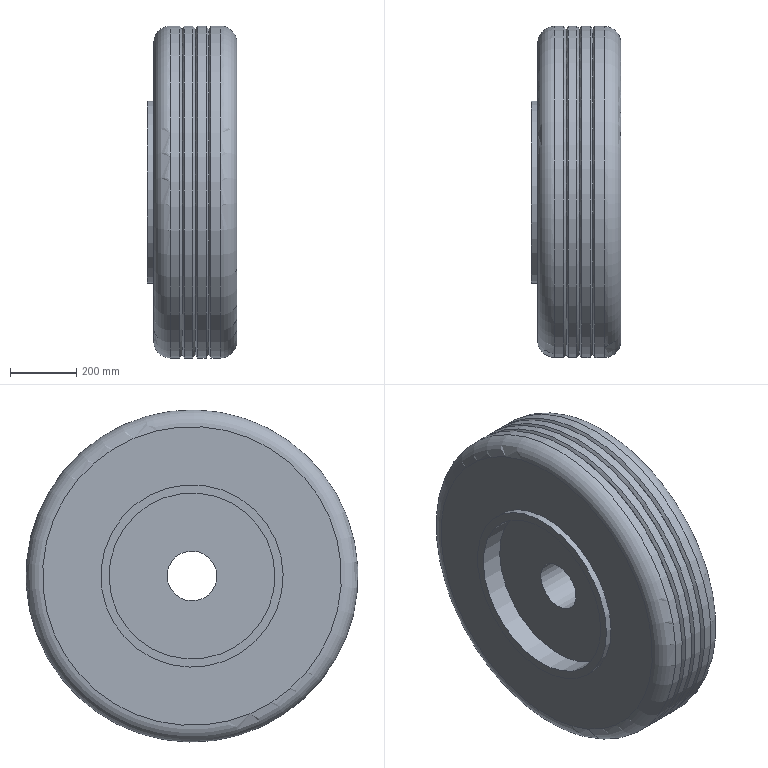Component | NX | WHEEL | 1 solid | 19 faces | box 270 x 1000 x 1000 mm | volume 179843524 mm3 | cylinder 7 | cone 6 | plane 4 | torus 2 | commonest cylinder face diameters 1000 x4 150 x1 500 x1 549 x1
STEP:
#1=CARTESIAN_POINT('',(0.,0.,0.));
#2=DIRECTION('',(0.,0.,1.));
#3=DIRECTION('',(1.,0.,0.));
#4=AXIS2_PLACEMENT_3D('',#1,#2,#3);
#5=CARTESIAN_POINT('',(283.134,-1440.025,-27.809));
#6=VERTEX_POINT('',#5);
#7=CARTESIAN_POINT('',(283.134,-1370.568,0.4891));
#8=DIRECTION('',(1.,0.,0.));
#9=DIRECTION('',(0.,-0.9261,-0.3773));
#10=AXIS2_PLACEMENT_3D('',#7,#8,#9);
#11=CIRCLE('',#10,75.);
#12=CARTESIAN_POINT('',(283.134,-1200.783,-416.252));
#13=DIRECTION('',(-1.,0.,0.));
#14=DIRECTION('',(0.,0.9261,0.3773));
#15=AXIS2_PLACEMENT_3D('',#12,#13,#14);
#16=PLANE('',#15);
#17=CARTESIAN_POINT('',(-75.,-450.));
#18=CARTESIAN_POINT('',(-75.,-320.096));
#19=CARTESIAN_POINT('',(37.5,-385.048));
#20=CARTESIAN_POINT('',(150.,-450.));
#21=CARTESIAN_POINT('',(37.5,-514.952));
#22=CARTESIAN_POINT('',(-75.,-579.904));
#23=CARTESIAN_POINT('',(-75.,-450.));
#24=(BOUNDED_CURVE()B_SPLINE_CURVE(2,(#17,#18,#19,#20,#21,#22,#23),.UNSPECIFIED.,.T.,.F.)B_SPLINE_CURVE_WITH_KNOTS((1,2,2,2,2,1),(-2.094,0.,2.094,4.189,6.283,8.378),.UNSPECIFIED.)CURVE()GEOMETRIC_REPRESENTATION_ITEM()RATIONAL_B_SPLINE_CURVE((1.,0.5,1.,0.5,1.,0.5,1.))REPRESENTATION_ITEM(''));
#25=(GEOMETRIC_REPRESENTATION_CONTEXT(2)PARAMETRIC_REPRESENTATION_CONTEXT()REPRESENTATION_CONTEXT('',''));
#26=DEFINITIONAL_REPRESENTATION('',(#24),#25);
#27=PCURVE('',#16,#26);
#28=CARTESIAN_POINT('',(158.134,-1370.568,0.4891));
#29=DIRECTION('',(1.,0.,0.));
#30=DIRECTION('',(0.,-0.9261,-0.3773));
#31=AXIS2_PLACEMENT_3D('',#28,#29,#30);
#32=CYLINDRICAL_SURFACE('',#31,75.);
#33=CARTESIAN_POINT('',(0.,125.));
#34=DIRECTION('',(1.,0.));
#35=VECTOR('',#34,1.);
#36=LINE('',#33,#35);
#37=(GEOMETRIC_REPRESENTATION_CONTEXT(2)PARAMETRIC_REPRESENTATION_CONTEXT()REPRESENTATION_CONTEXT('',''));
#38=DEFINITIONAL_REPRESENTATION('',(#36),#37);
#39=PCURVE('',#32,#38);
#40=SURFACE_CURVE('',#11,(#27,#39),.PCURVE_S1.);
#41=EDGE_CURVE('',#6,#6,#40,.T.);
#42=ORIENTED_EDGE('',*,*,#41,.F.);
#43=EDGE_LOOP('',(#42));
#44=FACE_BOUND('',#43,.T.);
#45=CARTESIAN_POINT('',(283.134,-1787.309,-169.297));
#46=VERTEX_POINT('',#45);
#47=CARTESIAN_POINT('',(283.134,-1370.568,0.4891));
#48=DIRECTION('',(1.,0.,0.));
#49=DIRECTION('',(0.,-0.9261,-0.3773));
#50=AXIS2_PLACEMENT_3D('',#47,#48,#49);
#51=CIRCLE('',#50,450.);
#52=CARTESIAN_POINT('',(-450.,-450.));
#53=CARTESIAN_POINT('',(-450.,329.423));
#54=CARTESIAN_POINT('',(225.,-60.289));
#55=CARTESIAN_POINT('',(900.,-450.));
#56=CARTESIAN_POINT('',(225.,-839.711));
#57=CARTESIAN_POINT('',(-450.,-1229.423));
#58=CARTESIAN_POINT('',(-450.,-450.));
#59=(BOUNDED_CURVE()B_SPLINE_CURVE(2,(#52,#53,#54,#55,#56,#57,#58),.UNSPECIFIED.,.T.,.F.)B_SPLINE_CURVE_WITH_KNOTS((1,2,2,2,2,1),(-2.094,0.,2.094,4.189,6.283,8.378),.UNSPECIFIED.)CURVE()GEOMETRIC_REPRESENTATION_ITEM()RATIONAL_B_SPLINE_CURVE((1.,0.5,1.,0.5,1.,0.5,1.))REPRESENTATION_ITEM(''));
#60=(GEOMETRIC_REPRESENTATION_CONTEXT(2)PARAMETRIC_REPRESENTATION_CONTEXT()REPRESENTATION_CONTEXT('',''));
#61=DEFINITIONAL_REPRESENTATION('',(#59),#60);
#62=PCURVE('',#16,#61);
#63=CARTESIAN_POINT('',(233.134,-1370.568,0.4891));
#64=DIRECTION('',(1.,0.,0.));
#65=DIRECTION('',(0.,-0.9261,-0.3773));
#66=AXIS2_PLACEMENT_3D('',#63,#64,#65);
#67=TOROIDAL_SURFACE('',#66,450.,50.);
#68=CARTESIAN_POINT('',(0.,7.854));
#69=DIRECTION('',(1.,0.));
#70=VECTOR('',#69,1.);
#71=LINE('',#68,#70);
#72=(GEOMETRIC_REPRESENTATION_CONTEXT(2)PARAMETRIC_REPRESENTATION_CONTEXT()REPRESENTATION_CONTEXT('',''));
#73=DEFINITIONAL_REPRESENTATION('',(#71),#72);
#74=PCURVE('',#67,#73);
#75=SURFACE_CURVE('',#51,(#62,#74),.PCURVE_S1.);
#76=EDGE_CURVE('',#46,#46,#75,.T.);
#77=ORIENTED_EDGE('',*,*,#76,.T.);
#78=EDGE_LOOP('',(#77));
#79=FACE_BOUND('',#78,.T.);
#80=ADVANCED_FACE('',(#44,#79),#16,.F.);
#81=CARTESIAN_POINT('',(83.134,-1440.025,-27.809));
#82=VERTEX_POINT('',#81);
#83=CARTESIAN_POINT('',(83.134,-1370.568,0.4891));
#84=DIRECTION('',(1.,0.,0.));
#85=DIRECTION('',(0.,-0.9261,-0.3773));
#86=AXIS2_PLACEMENT_3D('',#83,#84,#85);
#87=CIRCLE('',#86,75.);
#88=CARTESIAN_POINT('',(0.,-75.));
#89=DIRECTION('',(1.,0.));
#90=VECTOR('',#89,1.);
#91=LINE('',#88,#90);
#92=(GEOMETRIC_REPRESENTATION_CONTEXT(2)PARAMETRIC_REPRESENTATION_CONTEXT()REPRESENTATION_CONTEXT('',''));
#93=DEFINITIONAL_REPRESENTATION('',(#91),#92);
#94=PCURVE('',#32,#93);
#95=CARTESIAN_POINT('',(83.134,-1342.271,-68.968));
#96=DIRECTION('',(1.,0.,0.));
#97=DIRECTION('',(0.,-0.9261,-0.3773));
#98=AXIS2_PLACEMENT_3D('',#95,#96,#97);
#99=PLANE('',#98);
#100=CARTESIAN_POINT('',(-0.,-75.));
#101=DIRECTION('',(1.,0.));
#102=AXIS2_PLACEMENT_2D('',#100,#101);
#103=CIRCLE('',#102,75.);
#104=(GEOMETRIC_REPRESENTATION_CONTEXT(2)PARAMETRIC_REPRESENTATION_CONTEXT()REPRESENTATION_CONTEXT('',''));
#105=DEFINITIONAL_REPRESENTATION('',(#103),#104);
#106=PCURVE('',#99,#105);
#107=SURFACE_CURVE('',#87,(#94,#106),.PCURVE_S1.);
#108=EDGE_CURVE('',#82,#82,#107,.T.);
#109=ORIENTED_EDGE('',*,*,#108,.T.);
#110=CARTESIAN_POINT('',(83.134,-1440.025,-27.809));
#111=CARTESIAN_POINT('',(283.134,-1440.025,-27.809));
#112=B_SPLINE_CURVE_WITH_KNOTS('',1,(#110,#111),.UNSPECIFIED.,.F.,.F.,(2,2),(-75.,125.),.PIECEWISE_BEZIER_KNOTS.);
#113=CARTESIAN_POINT('',(6.283,0.));
#114=DIRECTION('',(0.,1.));
#115=VECTOR('',#114,1.);
#116=LINE('',#113,#115);
#117=(GEOMETRIC_REPRESENTATION_CONTEXT(2)PARAMETRIC_REPRESENTATION_CONTEXT()REPRESENTATION_CONTEXT('',''));
#118=DEFINITIONAL_REPRESENTATION('',(#116),#117);
#119=PCURVE('',#32,#118);
#120=CARTESIAN_POINT('',(0.,0.));
#121=DIRECTION('',(0.,1.));
#122=VECTOR('',#121,1.);
#123=LINE('',#120,#122);
#124=(GEOMETRIC_REPRESENTATION_CONTEXT(2)PARAMETRIC_REPRESENTATION_CONTEXT()REPRESENTATION_CONTEXT('',''));
#125=DEFINITIONAL_REPRESENTATION('',(#123),#124);
#126=PCURVE('',#32,#125);
#127=SEAM_CURVE('',#112,(#119,#126),.PCURVE_S1.);
#128=EDGE_CURVE('',#82,#6,#127,.T.);
#129=ORIENTED_EDGE('',*,*,#128,.T.);
#130=ORIENTED_EDGE('',*,*,#41,.F.);
#131=ORIENTED_EDGE('',*,*,#128,.F.);
#132=EDGE_LOOP('',(#109,#129,#130,#131));
#133=FACE_BOUND('',#132,.F.);
#134=ADVANCED_FACE('',(#133),#32,.F.);
#135=CARTESIAN_POINT('',(83.134,-1602.091,-93.836));
#136=VERTEX_POINT('',#135);
#137=CARTESIAN_POINT('',(83.134,-1370.568,0.4891));
#138=DIRECTION('',(1.,0.,0.));
#139=DIRECTION('',(0.,-0.9261,-0.3773));
#140=AXIS2_PLACEMENT_3D('',#137,#138,#139);
#141=CIRCLE('',#140,250.);
#142=CARTESIAN_POINT('',(-0.,-75.));
#143=DIRECTION('',(1.,0.));
#144=AXIS2_PLACEMENT_2D('',#142,#143);
#145=CIRCLE('',#144,250.);
#146=(GEOMETRIC_REPRESENTATION_CONTEXT(2)PARAMETRIC_REPRESENTATION_CONTEXT()REPRESENTATION_CONTEXT('',''));
#147=DEFINITIONAL_REPRESENTATION('',(#145),#146);
#148=PCURVE('',#99,#147);
#149=CARTESIAN_POINT('',(158.134,-1370.568,0.4891));
#150=DIRECTION('',(1.,0.,0.));
#151=DIRECTION('',(0.,-0.9261,-0.3773));
#152=AXIS2_PLACEMENT_3D('',#149,#150,#151);
#153=CYLINDRICAL_SURFACE('',#152,250.);
#154=CARTESIAN_POINT('',(0.,-75.));
#155=DIRECTION('',(1.,0.));
#156=VECTOR('',#155,1.);
#157=LINE('',#154,#156);
#158=(GEOMETRIC_REPRESENTATION_CONTEXT(2)PARAMETRIC_REPRESENTATION_CONTEXT()REPRESENTATION_CONTEXT('',''));
#159=DEFINITIONAL_REPRESENTATION('',(#157),#158);
#160=PCURVE('',#153,#159);
#161=SURFACE_CURVE('',#141,(#148,#160),.PCURVE_S1.);
#162=EDGE_CURVE('',#136,#136,#161,.T.);
#163=ORIENTED_EDGE('',*,*,#162,.F.);
#164=EDGE_LOOP('',(#163));
#165=FACE_BOUND('',#164,.T.);
#166=ORIENTED_EDGE('',*,*,#108,.T.);
#167=EDGE_LOOP('',(#166));
#168=FACE_BOUND('',#167,.T.);
#169=ADVANCED_FACE('',(#165,#168),#99,.F.);
#170=CARTESIAN_POINT('',(13.134,-1602.091,-93.836));
#171=VERTEX_POINT('',#170);
#172=CARTESIAN_POINT('',(13.134,-1370.568,0.4891));
#173=DIRECTION('',(1.,0.,0.));
#174=DIRECTION('',(0.,-0.9261,-0.3773));
#175=AXIS2_PLACEMENT_3D('',#172,#173,#174);
#176=CIRCLE('',#175,250.);
#177=CARTESIAN_POINT('',(0.,-145.));
#178=DIRECTION('',(1.,0.));
#179=VECTOR('',#178,1.);
#180=LINE('',#177,#179);
#181=(GEOMETRIC_REPRESENTATION_CONTEXT(2)PARAMETRIC_REPRESENTATION_CONTEXT()REPRESENTATION_CONTEXT('',''));
#182=DEFINITIONAL_REPRESENTATION('',(#180),#181);
#183=PCURVE('',#153,#182);
#184=CARTESIAN_POINT('',(13.134,-1276.243,-231.033));
#185=DIRECTION('',(1.,0.,0.));
#186=DIRECTION('',(0.,-0.9261,-0.3773));
#187=AXIS2_PLACEMENT_3D('',#184,#185,#186);
#188=PLANE('',#187);
#189=CARTESIAN_POINT('',(0.,-250.));
#190=DIRECTION('',(1.,0.));
#191=AXIS2_PLACEMENT_2D('',#189,#190);
#192=CIRCLE('',#191,250.);
#193=(GEOMETRIC_REPRESENTATION_CONTEXT(2)PARAMETRIC_REPRESENTATION_CONTEXT()REPRESENTATION_CONTEXT('',''));
#194=DEFINITIONAL_REPRESENTATION('',(#192),#193);
#195=PCURVE('',#188,#194);
#196=SURFACE_CURVE('',#176,(#183,#195),.PCURVE_S1.);
#197=EDGE_CURVE('',#171,#171,#196,.T.);
#198=ORIENTED_EDGE('',*,*,#197,.T.);
#199=CARTESIAN_POINT('',(13.134,-1602.091,-93.836));
#200=CARTESIAN_POINT('',(83.134,-1602.091,-93.836));
#201=B_SPLINE_CURVE_WITH_KNOTS('',1,(#199,#200),.UNSPECIFIED.,.F.,.F.,(2,2),(-145.,-75.),.PIECEWISE_BEZIER_KNOTS.);
#202=CARTESIAN_POINT('',(6.283,0.));
#203=DIRECTION('',(0.,1.));
#204=VECTOR('',#203,1.);
#205=LINE('',#202,#204);
#206=(GEOMETRIC_REPRESENTATION_CONTEXT(2)PARAMETRIC_REPRESENTATION_CONTEXT()REPRESENTATION_CONTEXT('',''));
#207=DEFINITIONAL_REPRESENTATION('',(#205),#206);
#208=PCURVE('',#153,#207);
#209=CARTESIAN_POINT('',(0.,0.));
#210=DIRECTION('',(0.,1.));
#211=VECTOR('',#210,1.);
#212=LINE('',#209,#211);
#213=(GEOMETRIC_REPRESENTATION_CONTEXT(2)PARAMETRIC_REPRESENTATION_CONTEXT()REPRESENTATION_CONTEXT('',''));
#214=DEFINITIONAL_REPRESENTATION('',(#212),#213);
#215=PCURVE('',#153,#214);
#216=SEAM_CURVE('',#201,(#208,#215),.PCURVE_S1.);
#217=EDGE_CURVE('',#171,#136,#216,.T.);
#218=ORIENTED_EDGE('',*,*,#217,.T.);
#219=ORIENTED_EDGE('',*,*,#162,.F.);
#220=ORIENTED_EDGE('',*,*,#217,.F.);
#221=EDGE_LOOP('',(#198,#218,#219,#220));
#222=FACE_BOUND('',#221,.F.);
#223=ADVANCED_FACE('',(#222),#153,.F.);
#224=CARTESIAN_POINT('',(13.134,-1624.78,-103.08));
#225=VERTEX_POINT('',#224);
#226=CARTESIAN_POINT('',(13.134,-1370.568,0.4891));
#227=DIRECTION('',(1.,0.,0.));
#228=DIRECTION('',(0.,-0.9261,-0.3773));
#229=AXIS2_PLACEMENT_3D('',#226,#227,#228);
#230=CIRCLE('',#229,274.5);
#231=CARTESIAN_POINT('',(0.,-250.));
#232=DIRECTION('',(1.,0.));
#233=AXIS2_PLACEMENT_2D('',#231,#232);
#234=CIRCLE('',#233,274.5);
#235=(GEOMETRIC_REPRESENTATION_CONTEXT(2)PARAMETRIC_REPRESENTATION_CONTEXT()REPRESENTATION_CONTEXT('',''));
#236=DEFINITIONAL_REPRESENTATION('',(#234),#235);
#237=PCURVE('',#188,#236);
#238=CARTESIAN_POINT('',(158.134,-1370.568,0.4891));
#239=DIRECTION('',(1.,0.,0.));
#240=DIRECTION('',(0.,-0.9261,-0.3773));
#241=AXIS2_PLACEMENT_3D('',#238,#239,#240);
#242=CYLINDRICAL_SURFACE('',#241,274.5);
#243=CARTESIAN_POINT('',(0.,-145.));
#244=DIRECTION('',(1.,0.));
#245=VECTOR('',#244,1.);
#246=LINE('',#243,#245);
#247=(GEOMETRIC_REPRESENTATION_CONTEXT(2)PARAMETRIC_REPRESENTATION_CONTEXT()REPRESENTATION_CONTEXT('',''));
#248=DEFINITIONAL_REPRESENTATION('',(#246),#247);
#249=PCURVE('',#242,#248);
#250=SURFACE_CURVE('',#230,(#237,#249),.PCURVE_S1.);
#251=EDGE_CURVE('',#225,#225,#250,.T.);
#252=ORIENTED_EDGE('',*,*,#251,.F.);
#253=EDGE_LOOP('',(#252));
#254=FACE_BOUND('',#253,.T.);
#255=ORIENTED_EDGE('',*,*,#197,.T.);
#256=EDGE_LOOP('',(#255));
#257=FACE_BOUND('',#256,.T.);
#258=ADVANCED_FACE('',(#254,#257),#188,.F.);
#259=CARTESIAN_POINT('',(33.134,-1624.78,-103.08));
#260=VERTEX_POINT('',#259);
#261=CARTESIAN_POINT('',(33.134,-1370.568,0.4891));
#262=DIRECTION('',(1.,0.,0.));
#263=DIRECTION('',(0.,-0.9261,-0.3773));
#264=AXIS2_PLACEMENT_3D('',#261,#262,#263);
#265=CIRCLE('',#264,274.5);
#266=CARTESIAN_POINT('',(0.,-125.));
#267=DIRECTION('',(1.,0.));
#268=VECTOR('',#267,1.);
#269=LINE('',#266,#268);
#270=(GEOMETRIC_REPRESENTATION_CONTEXT(2)PARAMETRIC_REPRESENTATION_CONTEXT()REPRESENTATION_CONTEXT('',''));
#271=DEFINITIONAL_REPRESENTATION('',(#269),#270);
#272=PCURVE('',#242,#271);
#273=CARTESIAN_POINT('',(33.134,-1266.999,-253.723));
#274=DIRECTION('',(1.,0.,0.));
#275=DIRECTION('',(0.,-0.9261,-0.3773));
#276=AXIS2_PLACEMENT_3D('',#273,#274,#275);
#277=PLANE('',#276);
#278=CARTESIAN_POINT('',(0.,-274.5));
#279=DIRECTION('',(1.,0.));
#280=AXIS2_PLACEMENT_2D('',#278,#279);
#281=CIRCLE('',#280,274.5);
#282=(GEOMETRIC_REPRESENTATION_CONTEXT(2)PARAMETRIC_REPRESENTATION_CONTEXT()REPRESENTATION_CONTEXT('',''));
#283=DEFINITIONAL_REPRESENTATION('',(#281),#282);
#284=PCURVE('',#277,#283);
#285=SURFACE_CURVE('',#265,(#272,#284),.PCURVE_S1.);
#286=EDGE_CURVE('',#260,#260,#285,.T.);
#287=ORIENTED_EDGE('',*,*,#286,.F.);
#288=CARTESIAN_POINT('',(13.134,-1624.78,-103.08));
#289=CARTESIAN_POINT('',(33.134,-1624.78,-103.08));
#290=B_SPLINE_CURVE_WITH_KNOTS('',1,(#288,#289),.UNSPECIFIED.,.F.,.F.,(2,2),(-145.,-125.),.PIECEWISE_BEZIER_KNOTS.);
#291=CARTESIAN_POINT('',(0.,0.));
#292=DIRECTION('',(0.,1.));
#293=VECTOR('',#292,1.);
#294=LINE('',#291,#293);
#295=(GEOMETRIC_REPRESENTATION_CONTEXT(2)PARAMETRIC_REPRESENTATION_CONTEXT()REPRESENTATION_CONTEXT('',''));
#296=DEFINITIONAL_REPRESENTATION('',(#294),#295);
#297=PCURVE('',#242,#296);
#298=CARTESIAN_POINT('',(6.283,0.));
#299=DIRECTION('',(0.,1.));
#300=VECTOR('',#299,1.);
#301=LINE('',#298,#300);
#302=(GEOMETRIC_REPRESENTATION_CONTEXT(2)PARAMETRIC_REPRESENTATION_CONTEXT()REPRESENTATION_CONTEXT('',''));
#303=DEFINITIONAL_REPRESENTATION('',(#301),#302);
#304=PCURVE('',#242,#303);
#305=SEAM_CURVE('',#290,(#297,#304),.PCURVE_S1.);
#306=EDGE_CURVE('',#225,#260,#305,.T.);
#307=ORIENTED_EDGE('',*,*,#306,.F.);
#308=ORIENTED_EDGE('',*,*,#251,.T.);
#309=ORIENTED_EDGE('',*,*,#306,.T.);
#310=EDGE_LOOP('',(#287,#307,#308,#309));
#311=FACE_BOUND('',#310,.T.);
#312=ADVANCED_FACE('',(#311),#242,.T.);
#313=CARTESIAN_POINT('',(33.134,-1787.309,-169.297));
#314=VERTEX_POINT('',#313);
#315=CARTESIAN_POINT('',(33.134,-1370.568,0.4891));
#316=DIRECTION('',(1.,0.,0.));
#317=DIRECTION('',(0.,-0.9261,-0.3773));
#318=AXIS2_PLACEMENT_3D('',#315,#316,#317);
#319=CIRCLE('',#318,450.);
#320=CARTESIAN_POINT('',(0.,-274.5));
#321=DIRECTION('',(1.,0.));
#322=AXIS2_PLACEMENT_2D('',#320,#321);
#323=CIRCLE('',#322,450.);
#324=(GEOMETRIC_REPRESENTATION_CONTEXT(2)PARAMETRIC_REPRESENTATION_CONTEXT()REPRESENTATION_CONTEXT('',''));
#325=DEFINITIONAL_REPRESENTATION('',(#323),#324);
#326=PCURVE('',#277,#325);
#327=CARTESIAN_POINT('',(83.134,-1370.568,0.4891));
#328=DIRECTION('',(1.,0.,0.));
#329=DIRECTION('',(0.,-0.9261,-0.3773));
#330=AXIS2_PLACEMENT_3D('',#327,#328,#329);
#331=TOROIDAL_SURFACE('',#330,450.,50.);
#332=CARTESIAN_POINT('',(0.,4.712));
#333=DIRECTION('',(1.,0.));
#334=VECTOR('',#333,1.);
#335=LINE('',#332,#334);
#336=(GEOMETRIC_REPRESENTATION_CONTEXT(2)PARAMETRIC_REPRESENTATION_CONTEXT()REPRESENTATION_CONTEXT('',''));
#337=DEFINITIONAL_REPRESENTATION('',(#335),#336);
#338=PCURVE('',#331,#337);
#339=SURFACE_CURVE('',#319,(#326,#338),.PCURVE_S1.);
#340=EDGE_CURVE('',#314,#314,#339,.T.);
#341=ORIENTED_EDGE('',*,*,#340,.F.);
#342=EDGE_LOOP('',(#341));
#343=FACE_BOUND('',#342,.T.);
#344=ORIENTED_EDGE('',*,*,#286,.T.);
#345=EDGE_LOOP('',(#344));
#346=FACE_BOUND('',#345,.T.);
#347=ADVANCED_FACE('',(#343,#346),#277,.F.);
#348=CARTESIAN_POINT('',(83.134,-1833.614,-188.162));
#349=VERTEX_POINT('',#348);
#350=CARTESIAN_POINT('',(83.134,-1370.568,0.4891));
#351=DIRECTION('',(1.,0.,0.));
#352=DIRECTION('',(0.,-0.9261,-0.3773));
#353=AXIS2_PLACEMENT_3D('',#350,#351,#352);
#354=CIRCLE('',#353,500.);
#355=CARTESIAN_POINT('',(0.,6.283));
#356=DIRECTION('',(1.,0.));
#357=VECTOR('',#356,1.);
#358=LINE('',#355,#357);
#359=(GEOMETRIC_REPRESENTATION_CONTEXT(2)PARAMETRIC_REPRESENTATION_CONTEXT()REPRESENTATION_CONTEXT('',''));
#360=DEFINITIONAL_REPRESENTATION('',(#358),#359);
#361=PCURVE('',#331,#360);
#362=CARTESIAN_POINT('',(158.134,-1370.568,0.4891));
#363=DIRECTION('',(1.,0.,0.));
#364=DIRECTION('',(0.,-0.9261,-0.3773));
#365=AXIS2_PLACEMENT_3D('',#362,#363,#364);
#366=CYLINDRICAL_SURFACE('',#365,500.);
#367=CARTESIAN_POINT('',(0.,-75.));
#368=DIRECTION('',(1.,0.));
#369=VECTOR('',#368,1.);
#370=LINE('',#367,#369);
#371=(GEOMETRIC_REPRESENTATION_CONTEXT(2)PARAMETRIC_REPRESENTATION_CONTEXT()REPRESENTATION_CONTEXT('',''));
#372=DEFINITIONAL_REPRESENTATION('',(#370),#371);
#373=PCURVE('',#366,#372);
#374=SURFACE_CURVE('',#354,(#361,#373),.PCURVE_S1.);
#375=EDGE_CURVE('',#349,#349,#374,.T.);
#376=ORIENTED_EDGE('',*,*,#375,.F.);
#377=CARTESIAN_POINT('',(33.134,-1787.309,-169.297));
#378=CARTESIAN_POINT('',(33.134,-1797.7,-173.53));
#379=CARTESIAN_POINT('',(36.071,-1808.09,-177.763));
#380=CARTESIAN_POINT('',(41.946,-1817.627,-181.649));
#381=CARTESIAN_POINT('',(50.396,-1825.453,-184.837));
#382=CARTESIAN_POINT('',(60.694,-1830.893,-187.054));
#383=CARTESIAN_POINT('',(71.914,-1833.614,-188.162));
#384=CARTESIAN_POINT('',(83.134,-1833.614,-188.162));
#385=B_SPLINE_CURVE_WITH_KNOTS('',7,(#377,#378,#379,#380,#381,#382,#383,#384),.UNSPECIFIED.,.F.,.F.,(8,8),(-1.571,0.),.PIECEWISE_BEZIER_KNOTS.);
#386=CARTESIAN_POINT('',(0.,6.283));
#387=DIRECTION('',(0.,1.));
#388=VECTOR('',#387,1.);
#389=LINE('',#386,#388);
#390=(GEOMETRIC_REPRESENTATION_CONTEXT(2)PARAMETRIC_REPRESENTATION_CONTEXT()REPRESENTATION_CONTEXT('',''));
#391=DEFINITIONAL_REPRESENTATION('',(#389),#390);
#392=PCURVE('',#331,#391);
#393=CARTESIAN_POINT('',(6.283,6.283));
#394=DIRECTION('',(0.,1.));
#395=VECTOR('',#394,1.);
#396=LINE('',#393,#395);
#397=(GEOMETRIC_REPRESENTATION_CONTEXT(2)PARAMETRIC_REPRESENTATION_CONTEXT()REPRESENTATION_CONTEXT('',''));
#398=DEFINITIONAL_REPRESENTATION('',(#396),#397);
#399=PCURVE('',#331,#398);
#400=SEAM_CURVE('',#385,(#392,#399),.PCURVE_S1.);
#401=EDGE_CURVE('',#314,#349,#400,.T.);
#402=ORIENTED_EDGE('',*,*,#401,.F.);
#403=ORIENTED_EDGE('',*,*,#340,.T.);
#404=ORIENTED_EDGE('',*,*,#401,.T.);
#405=EDGE_LOOP('',(#376,#402,#403,#404));
#406=FACE_BOUND('',#405,.T.);
#407=ADVANCED_FACE('',(#406),#331,.T.);
#408=CARTESIAN_POINT('',(110.746,-1833.614,-188.162));
#409=VERTEX_POINT('',#408);
#410=CARTESIAN_POINT('',(110.746,-1370.568,0.4891));
#411=DIRECTION('',(1.,0.,0.));
#412=DIRECTION('',(0.,-0.9261,-0.3773));
#413=AXIS2_PLACEMENT_3D('',#410,#411,#412);
#414=CIRCLE('',#413,500.);
#415=CARTESIAN_POINT('',(0.,-47.388));
#416=DIRECTION('',(1.,0.));
#417=VECTOR('',#416,1.);
#418=LINE('',#415,#417);
#419=(GEOMETRIC_REPRESENTATION_CONTEXT(2)PARAMETRIC_REPRESENTATION_CONTEXT()REPRESENTATION_CONTEXT('',''));
#420=DEFINITIONAL_REPRESENTATION('',(#418),#419);
#421=PCURVE('',#366,#420);
#422=CARTESIAN_POINT('',(110.746,-1370.568,0.4891));
#423=DIRECTION('',(-1.,0.,0.));
#424=DIRECTION('',(0.,0.9261,0.3773));
#425=AXIS2_PLACEMENT_3D('',#422,#423,#424);
#426=CONICAL_SURFACE('',#425,500.,0.925);
#427=CARTESIAN_POINT('',(9.425,0.));
#428=DIRECTION('',(-1.,0.));
#429=VECTOR('',#428,1.);
#430=LINE('',#427,#429);
#431=(GEOMETRIC_REPRESENTATION_CONTEXT(2)PARAMETRIC_REPRESENTATION_CONTEXT()REPRESENTATION_CONTEXT('',''));
#432=DEFINITIONAL_REPRESENTATION('',(#430),#431);
#433=PCURVE('',#426,#432);
#434=SURFACE_CURVE('',#414,(#421,#433),.PCURVE_S1.);
#435=EDGE_CURVE('',#409,#409,#434,.T.);
#436=ORIENTED_EDGE('',*,*,#435,.F.);
#437=CARTESIAN_POINT('',(83.134,-1833.614,-188.162));
#438=CARTESIAN_POINT('',(110.746,-1833.614,-188.162));
#439=B_SPLINE_CURVE_WITH_KNOTS('',1,(#437,#438),.UNSPECIFIED.,.F.,.F.,(2,2),(-75.,-47.388),.PIECEWISE_BEZIER_KNOTS.);
#440=CARTESIAN_POINT('',(0.,0.));
#441=DIRECTION('',(0.,1.));
#442=VECTOR('',#441,1.);
#443=LINE('',#440,#442);
#444=(GEOMETRIC_REPRESENTATION_CONTEXT(2)PARAMETRIC_REPRESENTATION_CONTEXT()REPRESENTATION_CONTEXT('',''));
#445=DEFINITIONAL_REPRESENTATION('',(#443),#444);
#446=PCURVE('',#366,#445);
#447=CARTESIAN_POINT('',(6.283,0.));
#448=DIRECTION('',(0.,1.));
#449=VECTOR('',#448,1.);
#450=LINE('',#447,#449);
#451=(GEOMETRIC_REPRESENTATION_CONTEXT(2)PARAMETRIC_REPRESENTATION_CONTEXT()REPRESENTATION_CONTEXT('',''));
#452=DEFINITIONAL_REPRESENTATION('',(#450),#451);
#453=PCURVE('',#366,#452);
#454=SEAM_CURVE('',#439,(#446,#453),.PCURVE_S1.);
#455=EDGE_CURVE('',#349,#409,#454,.T.);
#456=ORIENTED_EDGE('',*,*,#455,.F.);
#457=ORIENTED_EDGE('',*,*,#375,.T.);
#458=ORIENTED_EDGE('',*,*,#455,.T.);
#459=EDGE_LOOP('',(#436,#456,#457,#458));
#460=FACE_BOUND('',#459,.T.);
#461=ADVANCED_FACE('',(#460),#366,.T.);
#462=CARTESIAN_POINT('',(118.134,-1824.534,-184.463));
#463=VERTEX_POINT('',#462);
#464=CARTESIAN_POINT('',(118.134,-1370.568,0.4891));
#465=DIRECTION('',(1.,0.,0.));
#466=DIRECTION('',(0.,-0.9261,-0.3773));
#467=AXIS2_PLACEMENT_3D('',#464,#465,#466);
#468=CIRCLE('',#467,490.196);
#469=CARTESIAN_POINT('',(9.425,-7.388));
#470=DIRECTION('',(-1.,0.));
#471=VECTOR('',#470,1.);
#472=LINE('',#469,#471);
#473=(GEOMETRIC_REPRESENTATION_CONTEXT(2)PARAMETRIC_REPRESENTATION_CONTEXT()REPRESENTATION_CONTEXT('',''));
#474=DEFINITIONAL_REPRESENTATION('',(#472),#473);
#475=PCURVE('',#426,#474);
#476=CARTESIAN_POINT('',(118.134,-1370.568,0.4891));
#477=DIRECTION('',(1.,0.,0.));
#478=DIRECTION('',(0.,-0.9261,-0.3773));
#479=AXIS2_PLACEMENT_3D('',#476,#477,#478);
#480=CONICAL_SURFACE('',#479,490.196,0.9425);
#481=CARTESIAN_POINT('',(0.,0.));
#482=DIRECTION('',(1.,0.));
#483=VECTOR('',#482,1.);
#484=LINE('',#481,#483);
#485=(GEOMETRIC_REPRESENTATION_CONTEXT(2)PARAMETRIC_REPRESENTATION_CONTEXT()REPRESENTATION_CONTEXT('',''));
#486=DEFINITIONAL_REPRESENTATION('',(#484),#485);
#487=PCURVE('',#480,#486);
#488=SURFACE_CURVE('',#468,(#475,#487),.PCURVE_S1.);
#489=EDGE_CURVE('',#463,#463,#488,.T.);
#490=ORIENTED_EDGE('',*,*,#489,.F.);
#491=CARTESIAN_POINT('',(118.134,-1824.534,-184.463));
#492=CARTESIAN_POINT('',(110.746,-1833.614,-188.162));
#493=B_SPLINE_CURVE_WITH_KNOTS('',1,(#491,#492),.UNSPECIFIED.,.F.,.F.,(2,2),(-12.276,0.),.PIECEWISE_BEZIER_KNOTS.);
#494=CARTESIAN_POINT('',(9.425,0.));
#495=DIRECTION('',(0.,1.));
#496=VECTOR('',#495,1.);
#497=LINE('',#494,#496);
#498=(GEOMETRIC_REPRESENTATION_CONTEXT(2)PARAMETRIC_REPRESENTATION_CONTEXT()REPRESENTATION_CONTEXT('',''));
#499=DEFINITIONAL_REPRESENTATION('',(#497),#498);
#500=PCURVE('',#426,#499);
#501=CARTESIAN_POINT('',(3.142,0.));
#502=DIRECTION('',(0.,1.));
#503=VECTOR('',#502,1.);
#504=LINE('',#501,#503);
#505=(GEOMETRIC_REPRESENTATION_CONTEXT(2)PARAMETRIC_REPRESENTATION_CONTEXT()REPRESENTATION_CONTEXT('',''));
#506=DEFINITIONAL_REPRESENTATION('',(#504),#505);
#507=PCURVE('',#426,#506);
#508=SEAM_CURVE('',#493,(#500,#507),.PCURVE_S1.);
#509=EDGE_CURVE('',#463,#409,#508,.T.);
#510=ORIENTED_EDGE('',*,*,#509,.T.);
#511=ORIENTED_EDGE('',*,*,#435,.T.);
#512=ORIENTED_EDGE('',*,*,#509,.F.);
#513=EDGE_LOOP('',(#490,#510,#511,#512));
#514=FACE_BOUND('',#513,.T.);
#515=ADVANCED_FACE('',(#514),#426,.T.);
#516=CARTESIAN_POINT('',(125.257,-1833.614,-188.162));
#517=VERTEX_POINT('',#516);
#518=CARTESIAN_POINT('',(125.257,-1370.568,0.4891));
#519=DIRECTION('',(1.,0.,0.));
#520=DIRECTION('',(0.,-0.9261,-0.3773));
#521=AXIS2_PLACEMENT_3D('',#518,#519,#520);
#522=CIRCLE('',#521,500.);
#523=CARTESIAN_POINT('',(0.,7.123));
#524=DIRECTION('',(1.,0.));
#525=VECTOR('',#524,1.);
#526=LINE('',#523,#525);
#527=(GEOMETRIC_REPRESENTATION_CONTEXT(2)PARAMETRIC_REPRESENTATION_CONTEXT()REPRESENTATION_CONTEXT('',''));
#528=DEFINITIONAL_REPRESENTATION('',(#526),#527);
#529=PCURVE('',#480,#528);
#530=CARTESIAN_POINT('',(158.134,-1370.568,0.4891));
#531=DIRECTION('',(1.,0.,0.));
#532=DIRECTION('',(0.,-0.9261,-0.3773));
#533=AXIS2_PLACEMENT_3D('',#530,#531,#532);
#534=CYLINDRICAL_SURFACE('',#533,500.);
#535=CARTESIAN_POINT('',(0.,-32.877));
#536=DIRECTION('',(1.,0.));
#537=VECTOR('',#536,1.);
#538=LINE('',#535,#537);
#539=(GEOMETRIC_REPRESENTATION_CONTEXT(2)PARAMETRIC_REPRESENTATION_CONTEXT()REPRESENTATION_CONTEXT('',''));
#540=DEFINITIONAL_REPRESENTATION('',(#538),#539);
#541=PCURVE('',#534,#540);
#542=SURFACE_CURVE('',#522,(#529,#541),.PCURVE_S1.);
#543=EDGE_CURVE('',#517,#517,#542,.T.);
#544=ORIENTED_EDGE('',*,*,#543,.F.);
#545=CARTESIAN_POINT('',(118.134,-1824.534,-184.463));
#546=CARTESIAN_POINT('',(125.257,-1833.614,-188.162));
#547=B_SPLINE_CURVE_WITH_KNOTS('',1,(#545,#546),.UNSPECIFIED.,.F.,.F.,(2,2),(0.,12.118),.PIECEWISE_BEZIER_KNOTS.);
#548=CARTESIAN_POINT('',(0.,0.));
#549=DIRECTION('',(0.,1.));
#550=VECTOR('',#549,1.);
#551=LINE('',#548,#550);
#552=(GEOMETRIC_REPRESENTATION_CONTEXT(2)PARAMETRIC_REPRESENTATION_CONTEXT()REPRESENTATION_CONTEXT('',''));
#553=DEFINITIONAL_REPRESENTATION('',(#551),#552);
#554=PCURVE('',#480,#553);
#555=CARTESIAN_POINT('',(6.283,0.));
#556=DIRECTION('',(0.,1.));
#557=VECTOR('',#556,1.);
#558=LINE('',#555,#557);
#559=(GEOMETRIC_REPRESENTATION_CONTEXT(2)PARAMETRIC_REPRESENTATION_CONTEXT()REPRESENTATION_CONTEXT('',''));
#560=DEFINITIONAL_REPRESENTATION('',(#558),#559);
#561=PCURVE('',#480,#560);
#562=SEAM_CURVE('',#547,(#554,#561),.PCURVE_S1.);
#563=EDGE_CURVE('',#463,#517,#562,.T.);
#564=ORIENTED_EDGE('',*,*,#563,.F.);
#565=ORIENTED_EDGE('',*,*,#489,.T.);
#566=ORIENTED_EDGE('',*,*,#563,.T.);
#567=EDGE_LOOP('',(#544,#564,#565,#566));
#568=FACE_BOUND('',#567,.T.);
#569=ADVANCED_FACE('',(#568),#480,.T.);
#570=CARTESIAN_POINT('',(150.746,-1833.614,-188.162));
#571=VERTEX_POINT('',#570);
#572=CARTESIAN_POINT('',(150.746,-1370.568,0.4891));
#573=DIRECTION('',(1.,0.,0.));
#574=DIRECTION('',(0.,-0.9261,-0.3773));
#575=AXIS2_PLACEMENT_3D('',#572,#573,#574);
#576=CIRCLE('',#575,500.);
#577=CARTESIAN_POINT('',(0.,-7.388));
#578=DIRECTION('',(1.,0.));
#579=VECTOR('',#578,1.);
#580=LINE('',#577,#579);
#581=(GEOMETRIC_REPRESENTATION_CONTEXT(2)PARAMETRIC_REPRESENTATION_CONTEXT()REPRESENTATION_CONTEXT('',''));
#582=DEFINITIONAL_REPRESENTATION('',(#580),#581);
#583=PCURVE('',#534,#582);
#584=CARTESIAN_POINT('',(150.746,-1370.568,0.4891));
#585=DIRECTION('',(-1.,0.,0.));
#586=DIRECTION('',(0.,0.9261,0.3773));
#587=AXIS2_PLACEMENT_3D('',#584,#585,#586);
#588=CONICAL_SURFACE('',#587,500.,0.925);
#589=CARTESIAN_POINT('',(9.425,0.));
#590=DIRECTION('',(-1.,0.));
#591=VECTOR('',#590,1.);
#592=LINE('',#589,#591);
#593=(GEOMETRIC_REPRESENTATION_CONTEXT(2)PARAMETRIC_REPRESENTATION_CONTEXT()REPRESENTATION_CONTEXT('',''));
#594=DEFINITIONAL_REPRESENTATION('',(#592),#593);
#595=PCURVE('',#588,#594);
#596=SURFACE_CURVE('',#576,(#583,#595),.PCURVE_S1.);
#597=EDGE_CURVE('',#571,#571,#596,.T.);
#598=ORIENTED_EDGE('',*,*,#597,.F.);
#599=CARTESIAN_POINT('',(125.257,-1833.614,-188.162));
#600=CARTESIAN_POINT('',(150.746,-1833.614,-188.162));
#601=B_SPLINE_CURVE_WITH_KNOTS('',1,(#599,#600),.UNSPECIFIED.,.F.,.F.,(2,2),(-32.877,-7.388),.PIECEWISE_BEZIER_KNOTS.);
#602=CARTESIAN_POINT('',(0.,0.));
#603=DIRECTION('',(0.,1.));
#604=VECTOR('',#603,1.);
#605=LINE('',#602,#604);
#606=(GEOMETRIC_REPRESENTATION_CONTEXT(2)PARAMETRIC_REPRESENTATION_CONTEXT()REPRESENTATION_CONTEXT('',''));
#607=DEFINITIONAL_REPRESENTATION('',(#605),#606);
#608=PCURVE('',#534,#607);
#609=CARTESIAN_POINT('',(6.283,0.));
#610=DIRECTION('',(0.,1.));
#611=VECTOR('',#610,1.);
#612=LINE('',#609,#611);
#613=(GEOMETRIC_REPRESENTATION_CONTEXT(2)PARAMETRIC_REPRESENTATION_CONTEXT()REPRESENTATION_CONTEXT('',''));
#614=DEFINITIONAL_REPRESENTATION('',(#612),#613);
#615=PCURVE('',#534,#614);
#616=SEAM_CURVE('',#601,(#608,#615),.PCURVE_S1.);
#617=EDGE_CURVE('',#517,#571,#616,.T.);
#618=ORIENTED_EDGE('',*,*,#617,.F.);
#619=ORIENTED_EDGE('',*,*,#543,.T.);
#620=ORIENTED_EDGE('',*,*,#617,.T.);
#621=EDGE_LOOP('',(#598,#618,#619,#620));
#622=FACE_BOUND('',#621,.T.);
#623=ADVANCED_FACE('',(#622),#534,.T.);
#624=CARTESIAN_POINT('',(158.134,-1824.534,-184.463));
#625=VERTEX_POINT('',#624);
#626=CARTESIAN_POINT('',(158.134,-1370.568,0.4891));
#627=DIRECTION('',(1.,0.,0.));
#628=DIRECTION('',(0.,-0.9261,-0.3773));
#629=AXIS2_PLACEMENT_3D('',#626,#627,#628);
#630=CIRCLE('',#629,490.196);
#631=CARTESIAN_POINT('',(9.425,-7.388));
#632=DIRECTION('',(-1.,0.));
#633=VECTOR('',#632,1.);
#634=LINE('',#631,#633);
#635=(GEOMETRIC_REPRESENTATION_CONTEXT(2)PARAMETRIC_REPRESENTATION_CONTEXT()REPRESENTATION_CONTEXT('',''));
#636=DEFINITIONAL_REPRESENTATION('',(#634),#635);
#637=PCURVE('',#588,#636);
#638=CARTESIAN_POINT('',(158.134,-1370.568,0.4891));
#639=DIRECTION('',(1.,0.,0.));
#640=DIRECTION('',(0.,-0.9261,-0.3773));
#641=AXIS2_PLACEMENT_3D('',#638,#639,#640);
#642=CONICAL_SURFACE('',#641,490.196,0.9425);
#643=CARTESIAN_POINT('',(0.,0.));
#644=DIRECTION('',(1.,0.));
#645=VECTOR('',#644,1.);
#646=LINE('',#643,#645);
#647=(GEOMETRIC_REPRESENTATION_CONTEXT(2)PARAMETRIC_REPRESENTATION_CONTEXT()REPRESENTATION_CONTEXT('',''));
#648=DEFINITIONAL_REPRESENTATION('',(#646),#647);
#649=PCURVE('',#642,#648);
#650=SURFACE_CURVE('',#630,(#637,#649),.PCURVE_S1.);
#651=EDGE_CURVE('',#625,#625,#650,.T.);
#652=ORIENTED_EDGE('',*,*,#651,.F.);
#653=CARTESIAN_POINT('',(158.134,-1824.534,-184.463));
#654=CARTESIAN_POINT('',(150.746,-1833.614,-188.162));
#655=B_SPLINE_CURVE_WITH_KNOTS('',1,(#653,#654),.UNSPECIFIED.,.F.,.F.,(2,2),(-12.276,0.),.PIECEWISE_BEZIER_KNOTS.);
#656=CARTESIAN_POINT('',(9.425,0.));
#657=DIRECTION('',(0.,1.));
#658=VECTOR('',#657,1.);
#659=LINE('',#656,#658);
#660=(GEOMETRIC_REPRESENTATION_CONTEXT(2)PARAMETRIC_REPRESENTATION_CONTEXT()REPRESENTATION_CONTEXT('',''));
#661=DEFINITIONAL_REPRESENTATION('',(#659),#660);
#662=PCURVE('',#588,#661);
#663=CARTESIAN_POINT('',(3.142,0.));
#664=DIRECTION('',(0.,1.));
#665=VECTOR('',#664,1.);
#666=LINE('',#663,#665);
#667=(GEOMETRIC_REPRESENTATION_CONTEXT(2)PARAMETRIC_REPRESENTATION_CONTEXT()REPRESENTATION_CONTEXT('',''));
#668=DEFINITIONAL_REPRESENTATION('',(#666),#667);
#669=PCURVE('',#588,#668);
#670=SEAM_CURVE('',#655,(#662,#669),.PCURVE_S1.);
#671=EDGE_CURVE('',#625,#571,#670,.T.);
#672=ORIENTED_EDGE('',*,*,#671,.T.);
#673=ORIENTED_EDGE('',*,*,#597,.T.);
#674=ORIENTED_EDGE('',*,*,#671,.F.);
#675=EDGE_LOOP('',(#652,#672,#673,#674));
#676=FACE_BOUND('',#675,.T.);
#677=ADVANCED_FACE('',(#676),#588,.T.);
#678=CARTESIAN_POINT('',(165.257,-1833.614,-188.162));
#679=VERTEX_POINT('',#678);
#680=CARTESIAN_POINT('',(165.257,-1370.568,0.4891));
#681=DIRECTION('',(1.,0.,0.));
#682=DIRECTION('',(0.,-0.9261,-0.3773));
#683=AXIS2_PLACEMENT_3D('',#680,#681,#682);
#684=CIRCLE('',#683,500.);
#685=CARTESIAN_POINT('',(0.,7.123));
#686=DIRECTION('',(1.,0.));
#687=VECTOR('',#686,1.);
#688=LINE('',#685,#687);
#689=(GEOMETRIC_REPRESENTATION_CONTEXT(2)PARAMETRIC_REPRESENTATION_CONTEXT()REPRESENTATION_CONTEXT('',''));
#690=DEFINITIONAL_REPRESENTATION('',(#688),#689);
#691=PCURVE('',#642,#690);
#692=CARTESIAN_POINT('',(158.134,-1370.568,0.4891));
#693=DIRECTION('',(1.,0.,0.));
#694=DIRECTION('',(0.,-0.9261,-0.3773));
#695=AXIS2_PLACEMENT_3D('',#692,#693,#694);
#696=CYLINDRICAL_SURFACE('',#695,500.);
#697=CARTESIAN_POINT('',(0.,7.123));
#698=DIRECTION('',(1.,0.));
#699=VECTOR('',#698,1.);
#700=LINE('',#697,#699);
#701=(GEOMETRIC_REPRESENTATION_CONTEXT(2)PARAMETRIC_REPRESENTATION_CONTEXT()REPRESENTATION_CONTEXT('',''));
#702=DEFINITIONAL_REPRESENTATION('',(#700),#701);
#703=PCURVE('',#696,#702);
#704=SURFACE_CURVE('',#684,(#691,#703),.PCURVE_S1.);
#705=EDGE_CURVE('',#679,#679,#704,.T.);
#706=ORIENTED_EDGE('',*,*,#705,.F.);
#707=CARTESIAN_POINT('',(158.134,-1824.534,-184.463));
#708=CARTESIAN_POINT('',(165.257,-1833.614,-188.162));
#709=B_SPLINE_CURVE_WITH_KNOTS('',1,(#707,#708),.UNSPECIFIED.,.F.,.F.,(2,2),(0.,12.118),.PIECEWISE_BEZIER_KNOTS.);
#710=CARTESIAN_POINT('',(0.,0.));
#711=DIRECTION('',(0.,1.));
#712=VECTOR('',#711,1.);
#713=LINE('',#710,#712);
#714=(GEOMETRIC_REPRESENTATION_CONTEXT(2)PARAMETRIC_REPRESENTATION_CONTEXT()REPRESENTATION_CONTEXT('',''));
#715=DEFINITIONAL_REPRESENTATION('',(#713),#714);
#716=PCURVE('',#642,#715);
#717=CARTESIAN_POINT('',(6.283,0.));
#718=DIRECTION('',(0.,1.));
#719=VECTOR('',#718,1.);
#720=LINE('',#717,#719);
#721=(GEOMETRIC_REPRESENTATION_CONTEXT(2)PARAMETRIC_REPRESENTATION_CONTEXT()REPRESENTATION_CONTEXT('',''));
#722=DEFINITIONAL_REPRESENTATION('',(#720),#721);
#723=PCURVE('',#642,#722);
#724=SEAM_CURVE('',#709,(#716,#723),.PCURVE_S1.);
#725=EDGE_CURVE('',#625,#679,#724,.T.);
#726=ORIENTED_EDGE('',*,*,#725,.F.);
#727=ORIENTED_EDGE('',*,*,#651,.T.);
#728=ORIENTED_EDGE('',*,*,#725,.T.);
#729=EDGE_LOOP('',(#706,#726,#727,#728));
#730=FACE_BOUND('',#729,.T.);
#731=ADVANCED_FACE('',(#730),#642,.T.);
#732=CARTESIAN_POINT('',(190.746,-1833.614,-188.162));
#733=VERTEX_POINT('',#732);
#734=CARTESIAN_POINT('',(190.746,-1370.568,0.4891));
#735=DIRECTION('',(1.,0.,0.));
#736=DIRECTION('',(0.,-0.9261,-0.3773));
#737=AXIS2_PLACEMENT_3D('',#734,#735,#736);
#738=CIRCLE('',#737,500.);
#739=CARTESIAN_POINT('',(0.,32.612));
#740=DIRECTION('',(1.,0.));
#741=VECTOR('',#740,1.);
#742=LINE('',#739,#741);
#743=(GEOMETRIC_REPRESENTATION_CONTEXT(2)PARAMETRIC_REPRESENTATION_CONTEXT()REPRESENTATION_CONTEXT('',''));
#744=DEFINITIONAL_REPRESENTATION('',(#742),#743);
#745=PCURVE('',#696,#744);
#746=CARTESIAN_POINT('',(190.746,-1370.568,0.4891));
#747=DIRECTION('',(-1.,0.,0.));
#748=DIRECTION('',(0.,0.9261,0.3773));
#749=AXIS2_PLACEMENT_3D('',#746,#747,#748);
#750=CONICAL_SURFACE('',#749,500.,0.925);
#751=CARTESIAN_POINT('',(9.425,0.));
#752=DIRECTION('',(-1.,0.));
#753=VECTOR('',#752,1.);
#754=LINE('',#751,#753);
#755=(GEOMETRIC_REPRESENTATION_CONTEXT(2)PARAMETRIC_REPRESENTATION_CONTEXT()REPRESENTATION_CONTEXT('',''));
#756=DEFINITIONAL_REPRESENTATION('',(#754),#755);
#757=PCURVE('',#750,#756);
#758=SURFACE_CURVE('',#738,(#745,#757),.PCURVE_S1.);
#759=EDGE_CURVE('',#733,#733,#758,.T.);
#760=ORIENTED_EDGE('',*,*,#759,.F.);
#761=CARTESIAN_POINT('',(165.257,-1833.614,-188.162));
#762=CARTESIAN_POINT('',(190.746,-1833.614,-188.162));
#763=B_SPLINE_CURVE_WITH_KNOTS('',1,(#761,#762),.UNSPECIFIED.,.F.,.F.,(2,2),(7.123,32.612),.PIECEWISE_BEZIER_KNOTS.);
#764=CARTESIAN_POINT('',(0.,0.));
#765=DIRECTION('',(0.,1.));
#766=VECTOR('',#765,1.);
#767=LINE('',#764,#766);
#768=(GEOMETRIC_REPRESENTATION_CONTEXT(2)PARAMETRIC_REPRESENTATION_CONTEXT()REPRESENTATION_CONTEXT('',''));
#769=DEFINITIONAL_REPRESENTATION('',(#767),#768);
#770=PCURVE('',#696,#769);
#771=CARTESIAN_POINT('',(6.283,0.));
#772=DIRECTION('',(0.,1.));
#773=VECTOR('',#772,1.);
#774=LINE('',#771,#773);
#775=(GEOMETRIC_REPRESENTATION_CONTEXT(2)PARAMETRIC_REPRESENTATION_CONTEXT()REPRESENTATION_CONTEXT('',''));
#776=DEFINITIONAL_REPRESENTATION('',(#774),#775);
#777=PCURVE('',#696,#776);
#778=SEAM_CURVE('',#763,(#770,#777),.PCURVE_S1.);
#779=EDGE_CURVE('',#679,#733,#778,.T.);
#780=ORIENTED_EDGE('',*,*,#779,.F.);
#781=ORIENTED_EDGE('',*,*,#705,.T.);
#782=ORIENTED_EDGE('',*,*,#779,.T.);
#783=EDGE_LOOP('',(#760,#780,#781,#782));
#784=FACE_BOUND('',#783,.T.);
#785=ADVANCED_FACE('',(#784),#696,.T.);
#786=CARTESIAN_POINT('',(198.134,-1824.534,-184.463));
#787=VERTEX_POINT('',#786);
#788=CARTESIAN_POINT('',(198.134,-1370.568,0.4891));
#789=DIRECTION('',(1.,0.,0.));
#790=DIRECTION('',(0.,-0.9261,-0.3773));
#791=AXIS2_PLACEMENT_3D('',#788,#789,#790);
#792=CIRCLE('',#791,490.196);
#793=CARTESIAN_POINT('',(9.425,-7.388));
#794=DIRECTION('',(-1.,0.));
#795=VECTOR('',#794,1.);
#796=LINE('',#793,#795);
#797=(GEOMETRIC_REPRESENTATION_CONTEXT(2)PARAMETRIC_REPRESENTATION_CONTEXT()REPRESENTATION_CONTEXT('',''));
#798=DEFINITIONAL_REPRESENTATION('',(#796),#797);
#799=PCURVE('',#750,#798);
#800=CARTESIAN_POINT('',(198.134,-1370.568,0.4891));
#801=DIRECTION('',(1.,0.,0.));
#802=DIRECTION('',(0.,-0.9261,-0.3773));
#803=AXIS2_PLACEMENT_3D('',#800,#801,#802);
#804=CONICAL_SURFACE('',#803,490.196,0.9425);
#805=CARTESIAN_POINT('',(0.,0.));
#806=DIRECTION('',(1.,0.));
#807=VECTOR('',#806,1.);
#808=LINE('',#805,#807);
#809=(GEOMETRIC_REPRESENTATION_CONTEXT(2)PARAMETRIC_REPRESENTATION_CONTEXT()REPRESENTATION_CONTEXT('',''));
#810=DEFINITIONAL_REPRESENTATION('',(#808),#809);
#811=PCURVE('',#804,#810);
#812=SURFACE_CURVE('',#792,(#799,#811),.PCURVE_S1.);
#813=EDGE_CURVE('',#787,#787,#812,.T.);
#814=ORIENTED_EDGE('',*,*,#813,.F.);
#815=CARTESIAN_POINT('',(198.134,-1824.534,-184.463));
#816=CARTESIAN_POINT('',(190.746,-1833.614,-188.162));
#817=B_SPLINE_CURVE_WITH_KNOTS('',1,(#815,#816),.UNSPECIFIED.,.F.,.F.,(2,2),(-12.276,0.),.PIECEWISE_BEZIER_KNOTS.);
#818=CARTESIAN_POINT('',(9.425,0.));
#819=DIRECTION('',(0.,1.));
#820=VECTOR('',#819,1.);
#821=LINE('',#818,#820);
#822=(GEOMETRIC_REPRESENTATION_CONTEXT(2)PARAMETRIC_REPRESENTATION_CONTEXT()REPRESENTATION_CONTEXT('',''));
#823=DEFINITIONAL_REPRESENTATION('',(#821),#822);
#824=PCURVE('',#750,#823);
#825=CARTESIAN_POINT('',(3.142,0.));
#826=DIRECTION('',(0.,1.));
#827=VECTOR('',#826,1.);
#828=LINE('',#825,#827);
#829=(GEOMETRIC_REPRESENTATION_CONTEXT(2)PARAMETRIC_REPRESENTATION_CONTEXT()REPRESENTATION_CONTEXT('',''));
#830=DEFINITIONAL_REPRESENTATION('',(#828),#829);
#831=PCURVE('',#750,#830);
#832=SEAM_CURVE('',#817,(#824,#831),.PCURVE_S1.);
#833=EDGE_CURVE('',#787,#733,#832,.T.);
#834=ORIENTED_EDGE('',*,*,#833,.T.);
#835=ORIENTED_EDGE('',*,*,#759,.T.);
#836=ORIENTED_EDGE('',*,*,#833,.F.);
#837=EDGE_LOOP('',(#814,#834,#835,#836));
#838=FACE_BOUND('',#837,.T.);
#839=ADVANCED_FACE('',(#838),#750,.T.);
#840=CARTESIAN_POINT('',(205.257,-1833.614,-188.162));
#841=VERTEX_POINT('',#840);
#842=CARTESIAN_POINT('',(205.257,-1370.568,0.4891));
#843=DIRECTION('',(1.,0.,0.));
#844=DIRECTION('',(0.,-0.9261,-0.3773));
#845=AXIS2_PLACEMENT_3D('',#842,#843,#844);
#846=CIRCLE('',#845,500.);
#847=CARTESIAN_POINT('',(0.,7.123));
#848=DIRECTION('',(1.,0.));
#849=VECTOR('',#848,1.);
#850=LINE('',#847,#849);
#851=(GEOMETRIC_REPRESENTATION_CONTEXT(2)PARAMETRIC_REPRESENTATION_CONTEXT()REPRESENTATION_CONTEXT('',''));
#852=DEFINITIONAL_REPRESENTATION('',(#850),#851);
#853=PCURVE('',#804,#852);
#854=CARTESIAN_POINT('',(158.134,-1370.568,0.4891));
#855=DIRECTION('',(1.,0.,0.));
#856=DIRECTION('',(0.,-0.9261,-0.3773));
#857=AXIS2_PLACEMENT_3D('',#854,#855,#856);
#858=CYLINDRICAL_SURFACE('',#857,500.);
#859=CARTESIAN_POINT('',(0.,47.123));
#860=DIRECTION('',(1.,0.));
#861=VECTOR('',#860,1.);
#862=LINE('',#859,#861);
#863=(GEOMETRIC_REPRESENTATION_CONTEXT(2)PARAMETRIC_REPRESENTATION_CONTEXT()REPRESENTATION_CONTEXT('',''));
#864=DEFINITIONAL_REPRESENTATION('',(#862),#863);
#865=PCURVE('',#858,#864);
#866=SURFACE_CURVE('',#846,(#853,#865),.PCURVE_S1.);
#867=EDGE_CURVE('',#841,#841,#866,.T.);
#868=ORIENTED_EDGE('',*,*,#867,.F.);
#869=CARTESIAN_POINT('',(198.134,-1824.534,-184.463));
#870=CARTESIAN_POINT('',(205.257,-1833.614,-188.162));
#871=B_SPLINE_CURVE_WITH_KNOTS('',1,(#869,#870),.UNSPECIFIED.,.F.,.F.,(2,2),(0.,12.118),.PIECEWISE_BEZIER_KNOTS.);
#872=CARTESIAN_POINT('',(0.,0.));
#873=DIRECTION('',(0.,1.));
#874=VECTOR('',#873,1.);
#875=LINE('',#872,#874);
#876=(GEOMETRIC_REPRESENTATION_CONTEXT(2)PARAMETRIC_REPRESENTATION_CONTEXT()REPRESENTATION_CONTEXT('',''));
#877=DEFINITIONAL_REPRESENTATION('',(#875),#876);
#878=PCURVE('',#804,#877);
#879=CARTESIAN_POINT('',(6.283,0.));
#880=DIRECTION('',(0.,1.));
#881=VECTOR('',#880,1.);
#882=LINE('',#879,#881);
#883=(GEOMETRIC_REPRESENTATION_CONTEXT(2)PARAMETRIC_REPRESENTATION_CONTEXT()REPRESENTATION_CONTEXT('',''));
#884=DEFINITIONAL_REPRESENTATION('',(#882),#883);
#885=PCURVE('',#804,#884);
#886=SEAM_CURVE('',#871,(#878,#885),.PCURVE_S1.);
#887=EDGE_CURVE('',#787,#841,#886,.T.);
#888=ORIENTED_EDGE('',*,*,#887,.F.);
#889=ORIENTED_EDGE('',*,*,#813,.T.);
#890=ORIENTED_EDGE('',*,*,#887,.T.);
#891=EDGE_LOOP('',(#868,#888,#889,#890));
#892=FACE_BOUND('',#891,.T.);
#893=ADVANCED_FACE('',(#892),#804,.T.);
#894=CARTESIAN_POINT('',(233.134,-1833.614,-188.162));
#895=VERTEX_POINT('',#894);
#896=CARTESIAN_POINT('',(233.134,-1370.568,0.4891));
#897=DIRECTION('',(1.,0.,0.));
#898=DIRECTION('',(0.,-0.9261,-0.3773));
#899=AXIS2_PLACEMENT_3D('',#896,#897,#898);
#900=CIRCLE('',#899,500.);
#901=CARTESIAN_POINT('',(0.,75.));
#902=DIRECTION('',(1.,0.));
#903=VECTOR('',#902,1.);
#904=LINE('',#901,#903);
#905=(GEOMETRIC_REPRESENTATION_CONTEXT(2)PARAMETRIC_REPRESENTATION_CONTEXT()REPRESENTATION_CONTEXT('',''));
#906=DEFINITIONAL_REPRESENTATION('',(#904),#905);
#907=PCURVE('',#858,#906);
#908=CARTESIAN_POINT('',(0.,6.283));
#909=DIRECTION('',(1.,0.));
#910=VECTOR('',#909,1.);
#911=LINE('',#908,#910);
#912=(GEOMETRIC_REPRESENTATION_CONTEXT(2)PARAMETRIC_REPRESENTATION_CONTEXT()REPRESENTATION_CONTEXT('',''));
#913=DEFINITIONAL_REPRESENTATION('',(#911),#912);
#914=PCURVE('',#67,#913);
#915=SURFACE_CURVE('',#900,(#907,#914),.PCURVE_S1.);
#916=EDGE_CURVE('',#895,#895,#915,.T.);
#917=ORIENTED_EDGE('',*,*,#916,.F.);
#918=CARTESIAN_POINT('',(205.257,-1833.614,-188.162));
#919=CARTESIAN_POINT('',(233.134,-1833.614,-188.162));
#920=B_SPLINE_CURVE_WITH_KNOTS('',1,(#918,#919),.UNSPECIFIED.,.F.,.F.,(2,2),(47.123,75.),.PIECEWISE_BEZIER_KNOTS.);
#921=CARTESIAN_POINT('',(0.,0.));
#922=DIRECTION('',(0.,1.));
#923=VECTOR('',#922,1.);
#924=LINE('',#921,#923);
#925=(GEOMETRIC_REPRESENTATION_CONTEXT(2)PARAMETRIC_REPRESENTATION_CONTEXT()REPRESENTATION_CONTEXT('',''));
#926=DEFINITIONAL_REPRESENTATION('',(#924),#925);
#927=PCURVE('',#858,#926);
#928=CARTESIAN_POINT('',(6.283,0.));
#929=DIRECTION('',(0.,1.));
#930=VECTOR('',#929,1.);
#931=LINE('',#928,#930);
#932=(GEOMETRIC_REPRESENTATION_CONTEXT(2)PARAMETRIC_REPRESENTATION_CONTEXT()REPRESENTATION_CONTEXT('',''));
#933=DEFINITIONAL_REPRESENTATION('',(#931),#932);
#934=PCURVE('',#858,#933);
#935=SEAM_CURVE('',#920,(#927,#934),.PCURVE_S1.);
#936=EDGE_CURVE('',#841,#895,#935,.T.);
#937=ORIENTED_EDGE('',*,*,#936,.F.);
#938=ORIENTED_EDGE('',*,*,#867,.T.);
#939=ORIENTED_EDGE('',*,*,#936,.T.);
#940=EDGE_LOOP('',(#917,#937,#938,#939));
#941=FACE_BOUND('',#940,.T.);
#942=ADVANCED_FACE('',(#941),#858,.T.);
#943=ORIENTED_EDGE('',*,*,#76,.F.);
#944=CARTESIAN_POINT('',(233.134,-1833.614,-188.162));
#945=CARTESIAN_POINT('',(244.354,-1833.614,-188.162));
#946=CARTESIAN_POINT('',(255.574,-1830.893,-187.054));
#947=CARTESIAN_POINT('',(265.871,-1825.453,-184.837));
#948=CARTESIAN_POINT('',(274.322,-1817.627,-181.649));
#949=CARTESIAN_POINT('',(280.196,-1808.09,-177.763));
#950=CARTESIAN_POINT('',(283.134,-1797.7,-173.53));
#951=CARTESIAN_POINT('',(283.134,-1787.309,-169.297));
#952=B_SPLINE_CURVE_WITH_KNOTS('',7,(#944,#945,#946,#947,#948,#949,#950,#951),.UNSPECIFIED.,.F.,.F.,(8,8),(0.,1.571),.PIECEWISE_BEZIER_KNOTS.);
#953=CARTESIAN_POINT('',(0.,6.283));
#954=DIRECTION('',(0.,1.));
#955=VECTOR('',#954,1.);
#956=LINE('',#953,#955);
#957=(GEOMETRIC_REPRESENTATION_CONTEXT(2)PARAMETRIC_REPRESENTATION_CONTEXT()REPRESENTATION_CONTEXT('',''));
#958=DEFINITIONAL_REPRESENTATION('',(#956),#957);
#959=PCURVE('',#67,#958);
#960=CARTESIAN_POINT('',(6.283,6.283));
#961=DIRECTION('',(0.,1.));
#962=VECTOR('',#961,1.);
#963=LINE('',#960,#962);
#964=(GEOMETRIC_REPRESENTATION_CONTEXT(2)PARAMETRIC_REPRESENTATION_CONTEXT()REPRESENTATION_CONTEXT('',''));
#965=DEFINITIONAL_REPRESENTATION('',(#963),#964);
#966=PCURVE('',#67,#965);
#967=SEAM_CURVE('',#952,(#959,#966),.PCURVE_S1.);
#968=EDGE_CURVE('',#895,#46,#967,.T.);
#969=ORIENTED_EDGE('',*,*,#968,.F.);
#970=ORIENTED_EDGE('',*,*,#916,.T.);
#971=ORIENTED_EDGE('',*,*,#968,.T.);
#972=EDGE_LOOP('',(#943,#969,#970,#971));
#973=FACE_BOUND('',#972,.T.);
#974=ADVANCED_FACE('',(#973),#67,.T.);
#975=CLOSED_SHELL('',(#80,#134,#169,#223,#258,#312,#347,#407,#461,#515,#569,#623,#677,#731,#785,#839,#893,#942,#974));
#976=MANIFOLD_SOLID_BREP('',#975);
#977=(LENGTH_UNIT()NAMED_UNIT(*)SI_UNIT(.MILLI.,.METRE.));
#978=UNCERTAINTY_MEASURE_WITH_UNIT(LENGTH_MEASURE(0.00001),#977,'','');
#979=(NAMED_UNIT(*)PLANE_ANGLE_UNIT()SI_UNIT($,.RADIAN.));
#980=(NAMED_UNIT(*)SI_UNIT($,.STERADIAN.)SOLID_ANGLE_UNIT());
#981=(GEOMETRIC_REPRESENTATION_CONTEXT(3)GLOBAL_UNCERTAINTY_ASSIGNED_CONTEXT((#978))GLOBAL_UNIT_ASSIGNED_CONTEXT((#977,#979,#980))REPRESENTATION_CONTEXT('',''));
#982=ADVANCED_BREP_SHAPE_REPRESENTATION('',(#4,#976),#981);